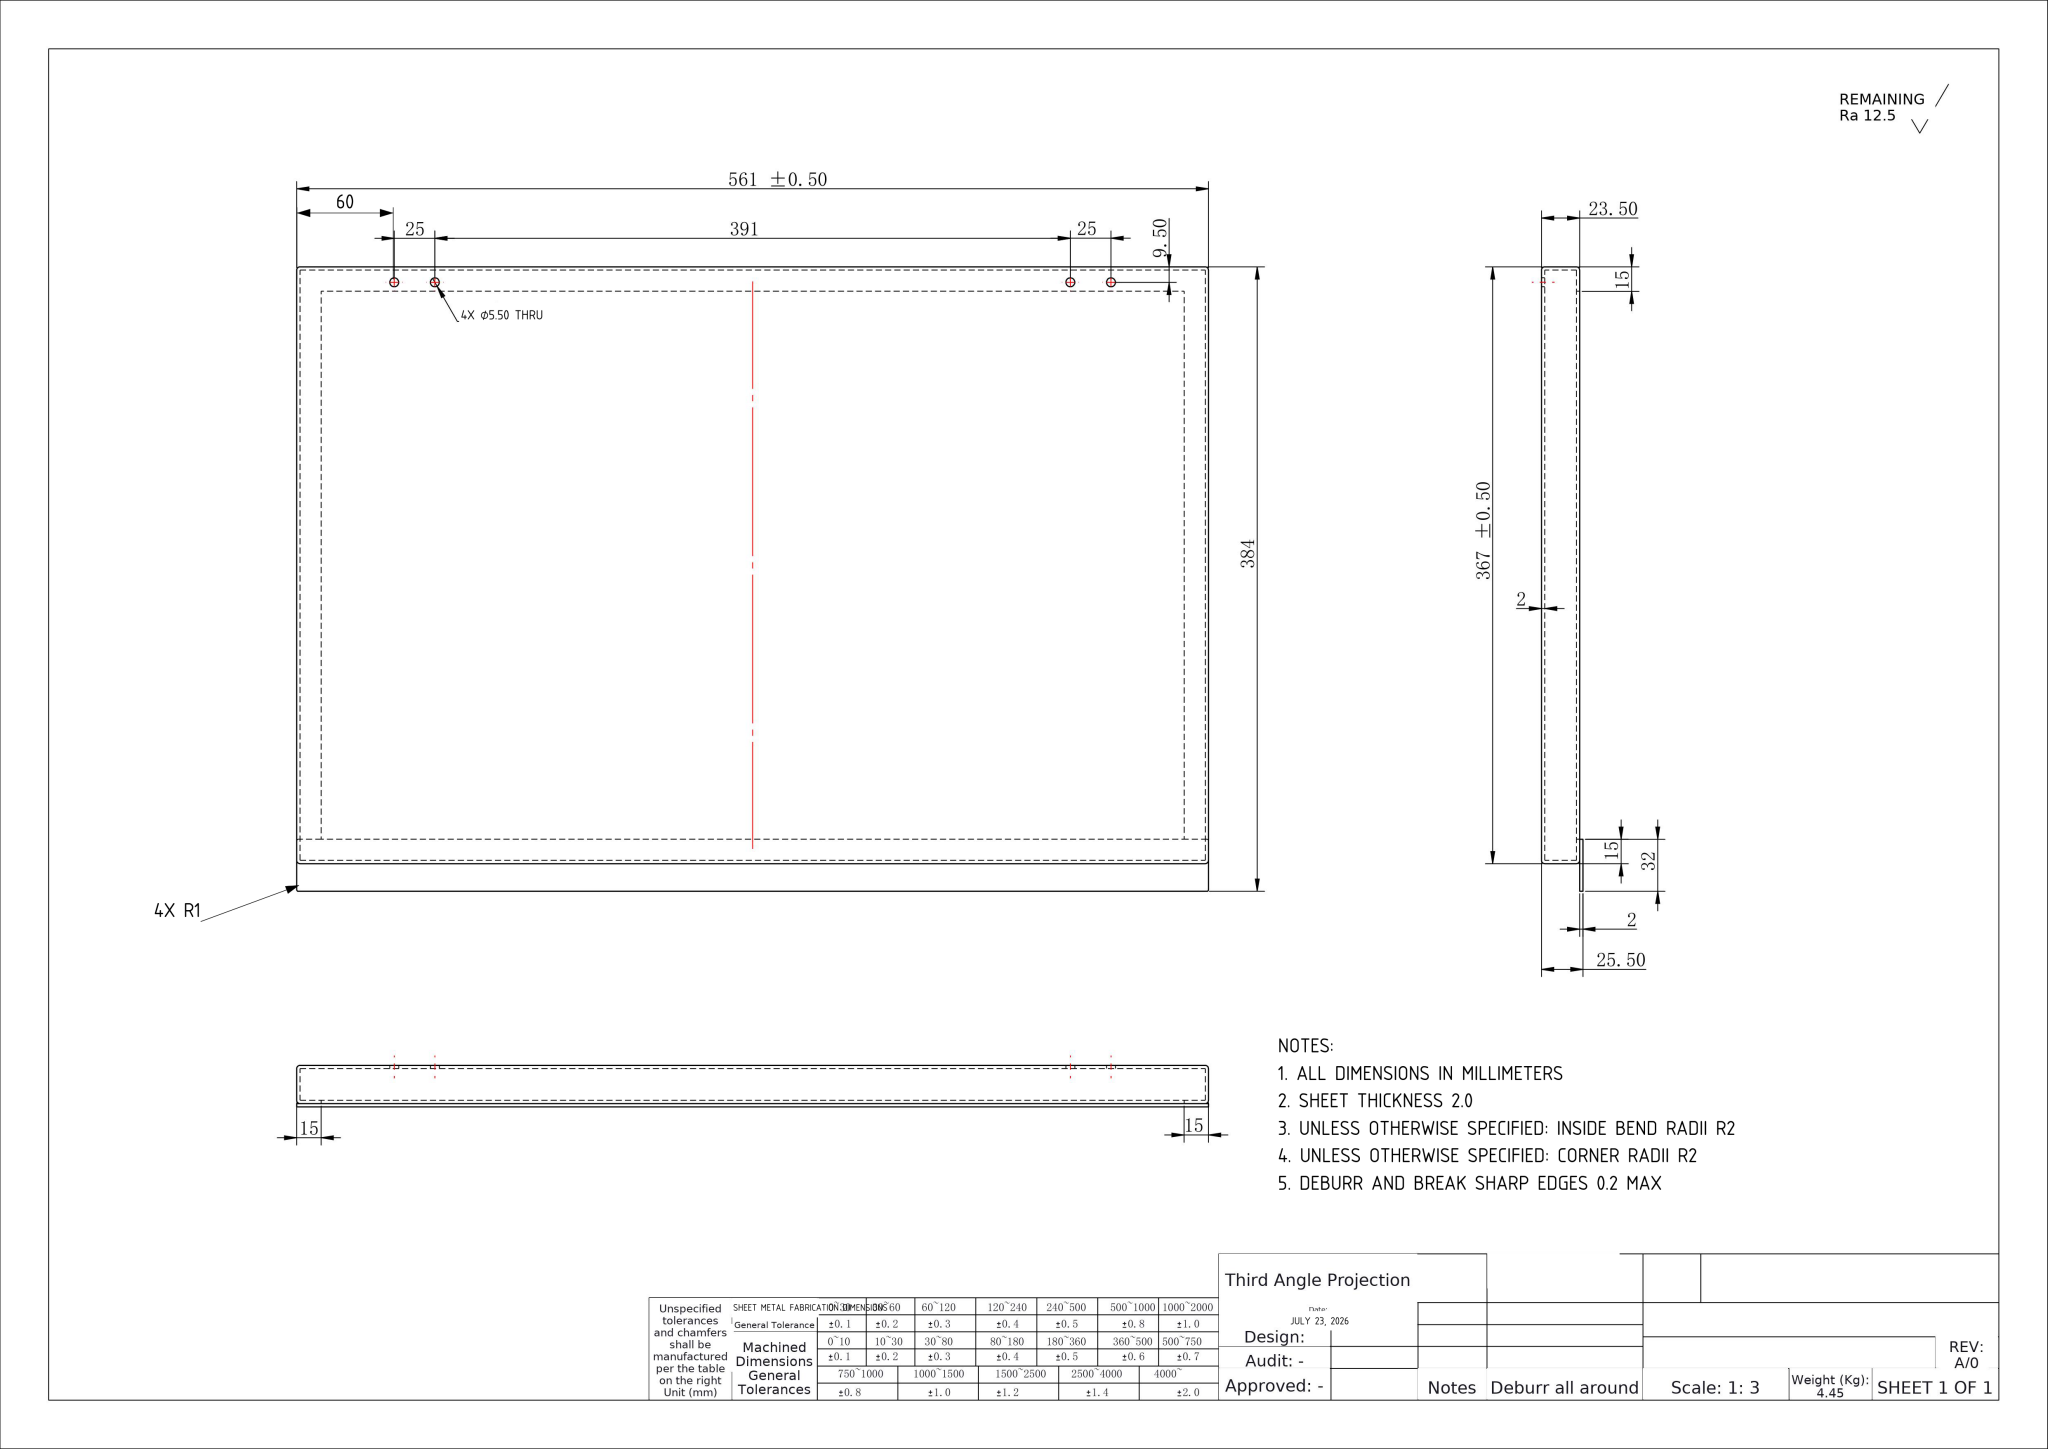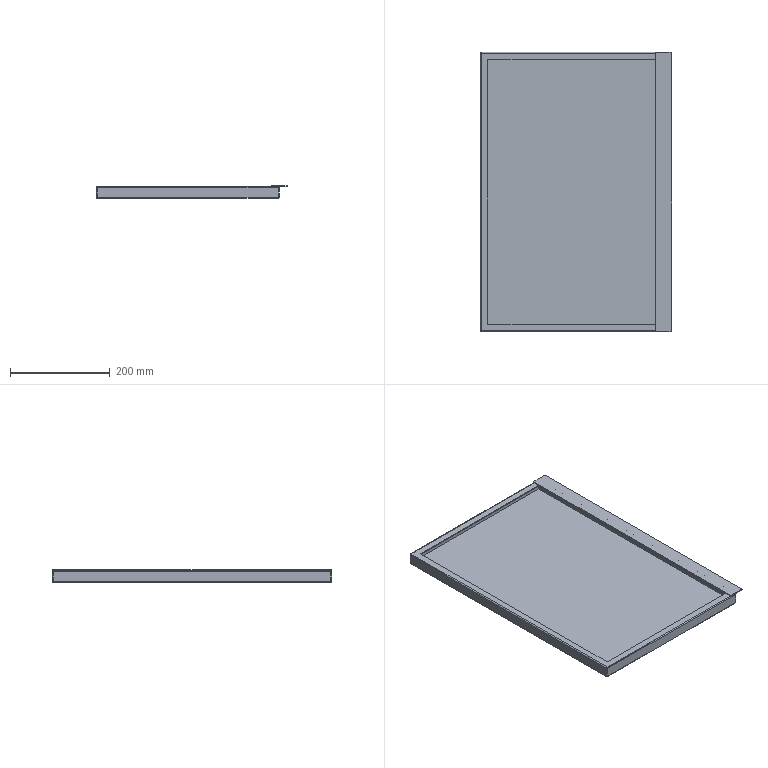Part | NX | mm | 1 solid | 53 faces | box 384 x 561 x 25.5 mm | volume 570182 mm3 | cylinder 24 | plane 21 | sphere 8 | commonest cylinder face diameters 4 x12 5.5 x8 2 x4